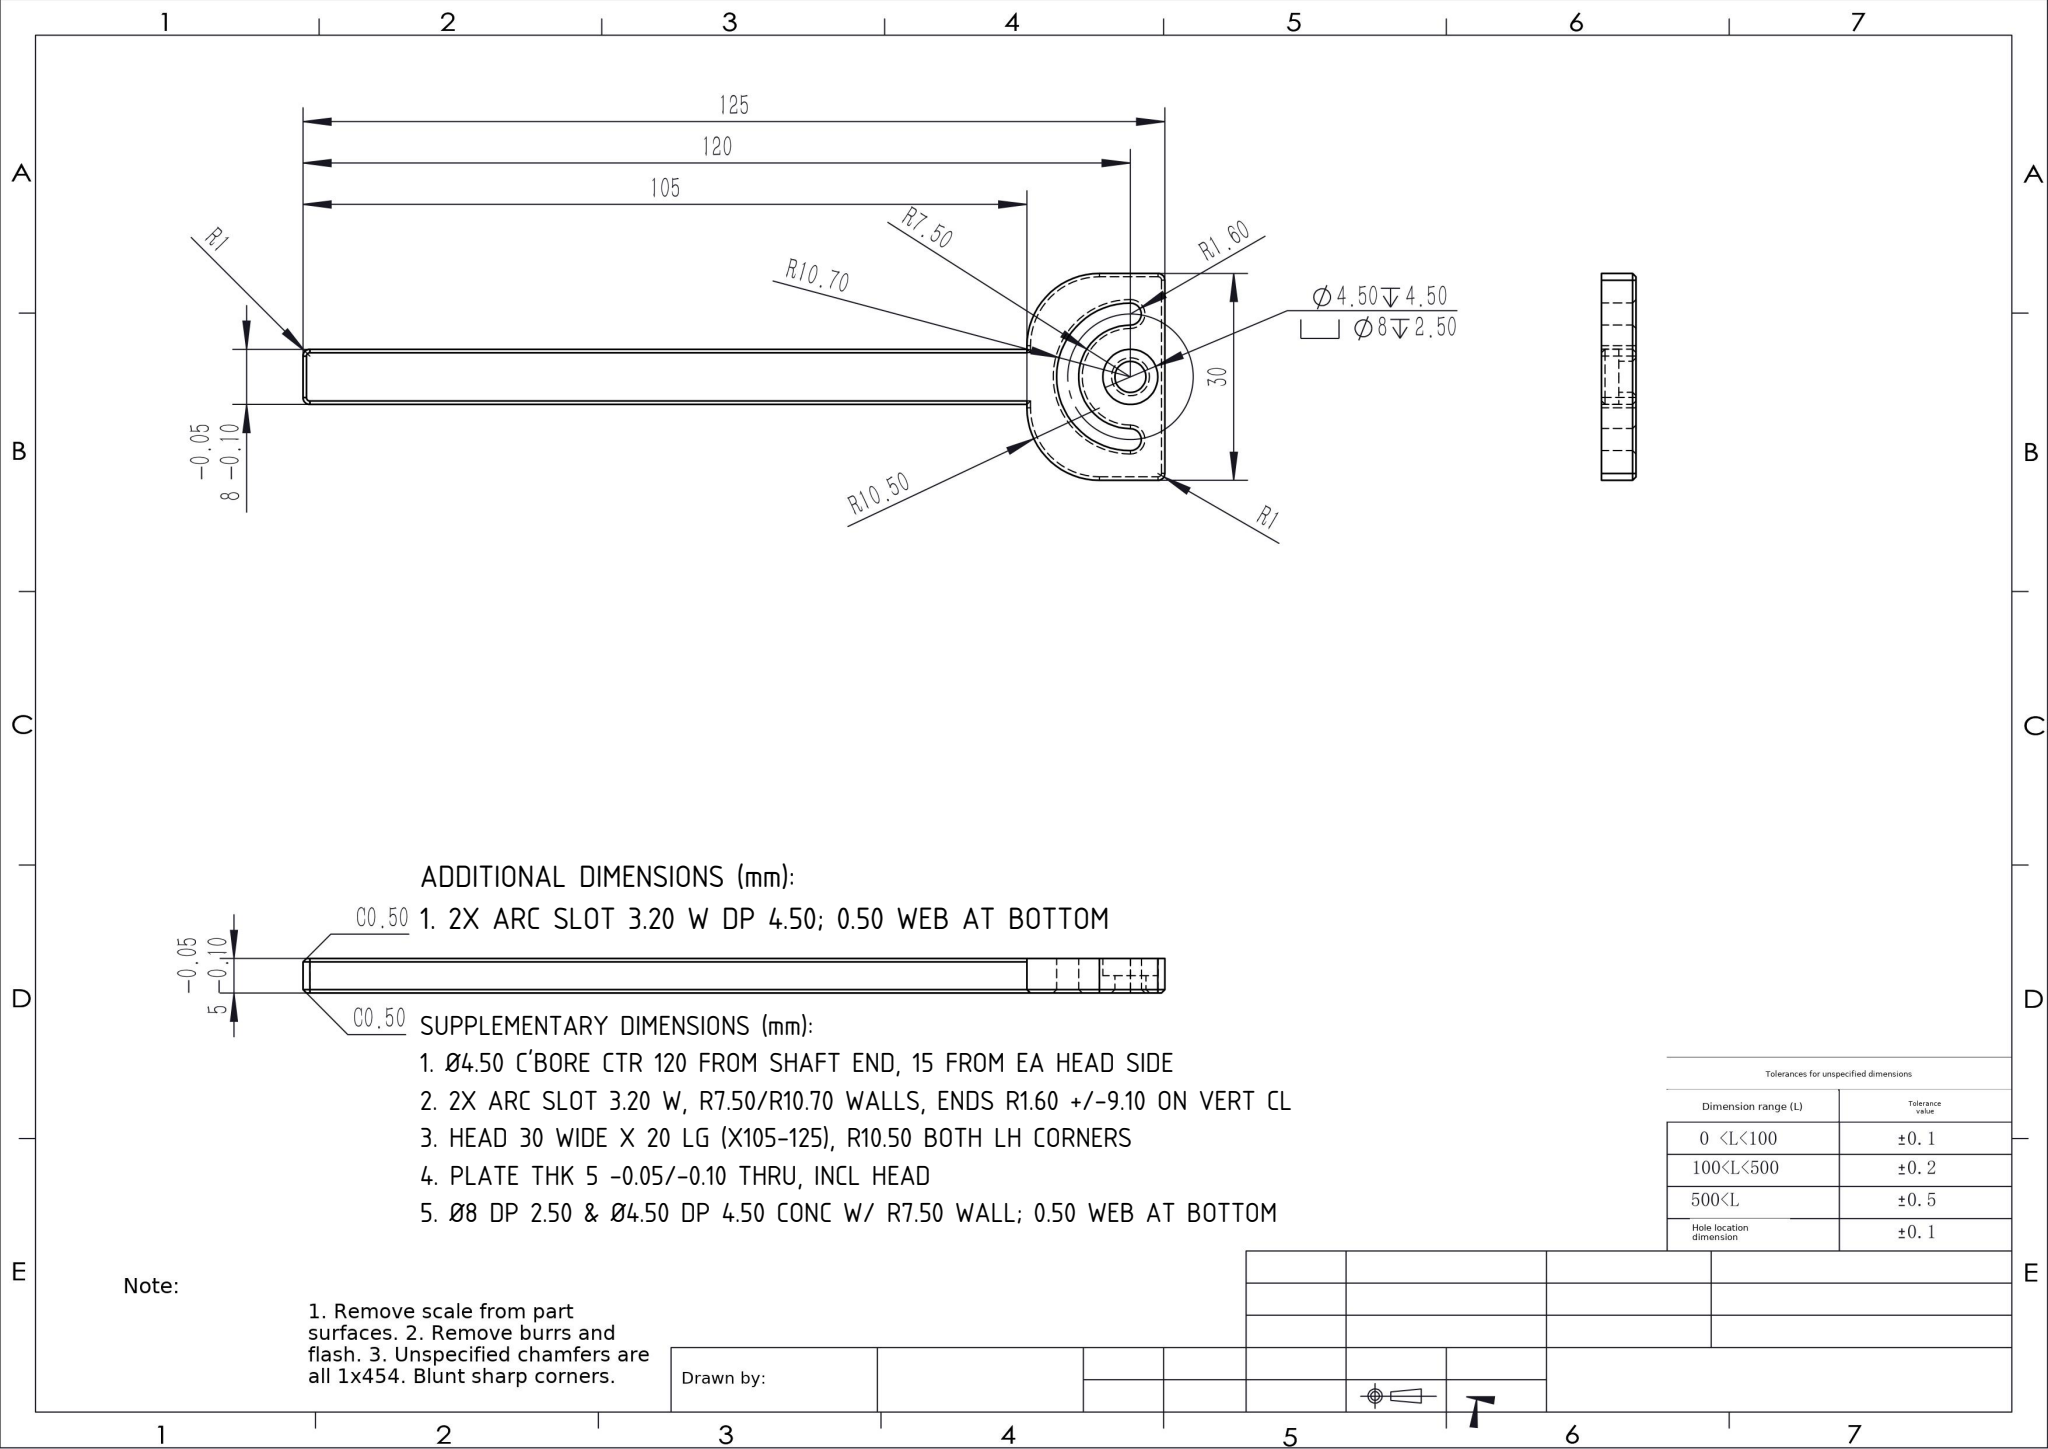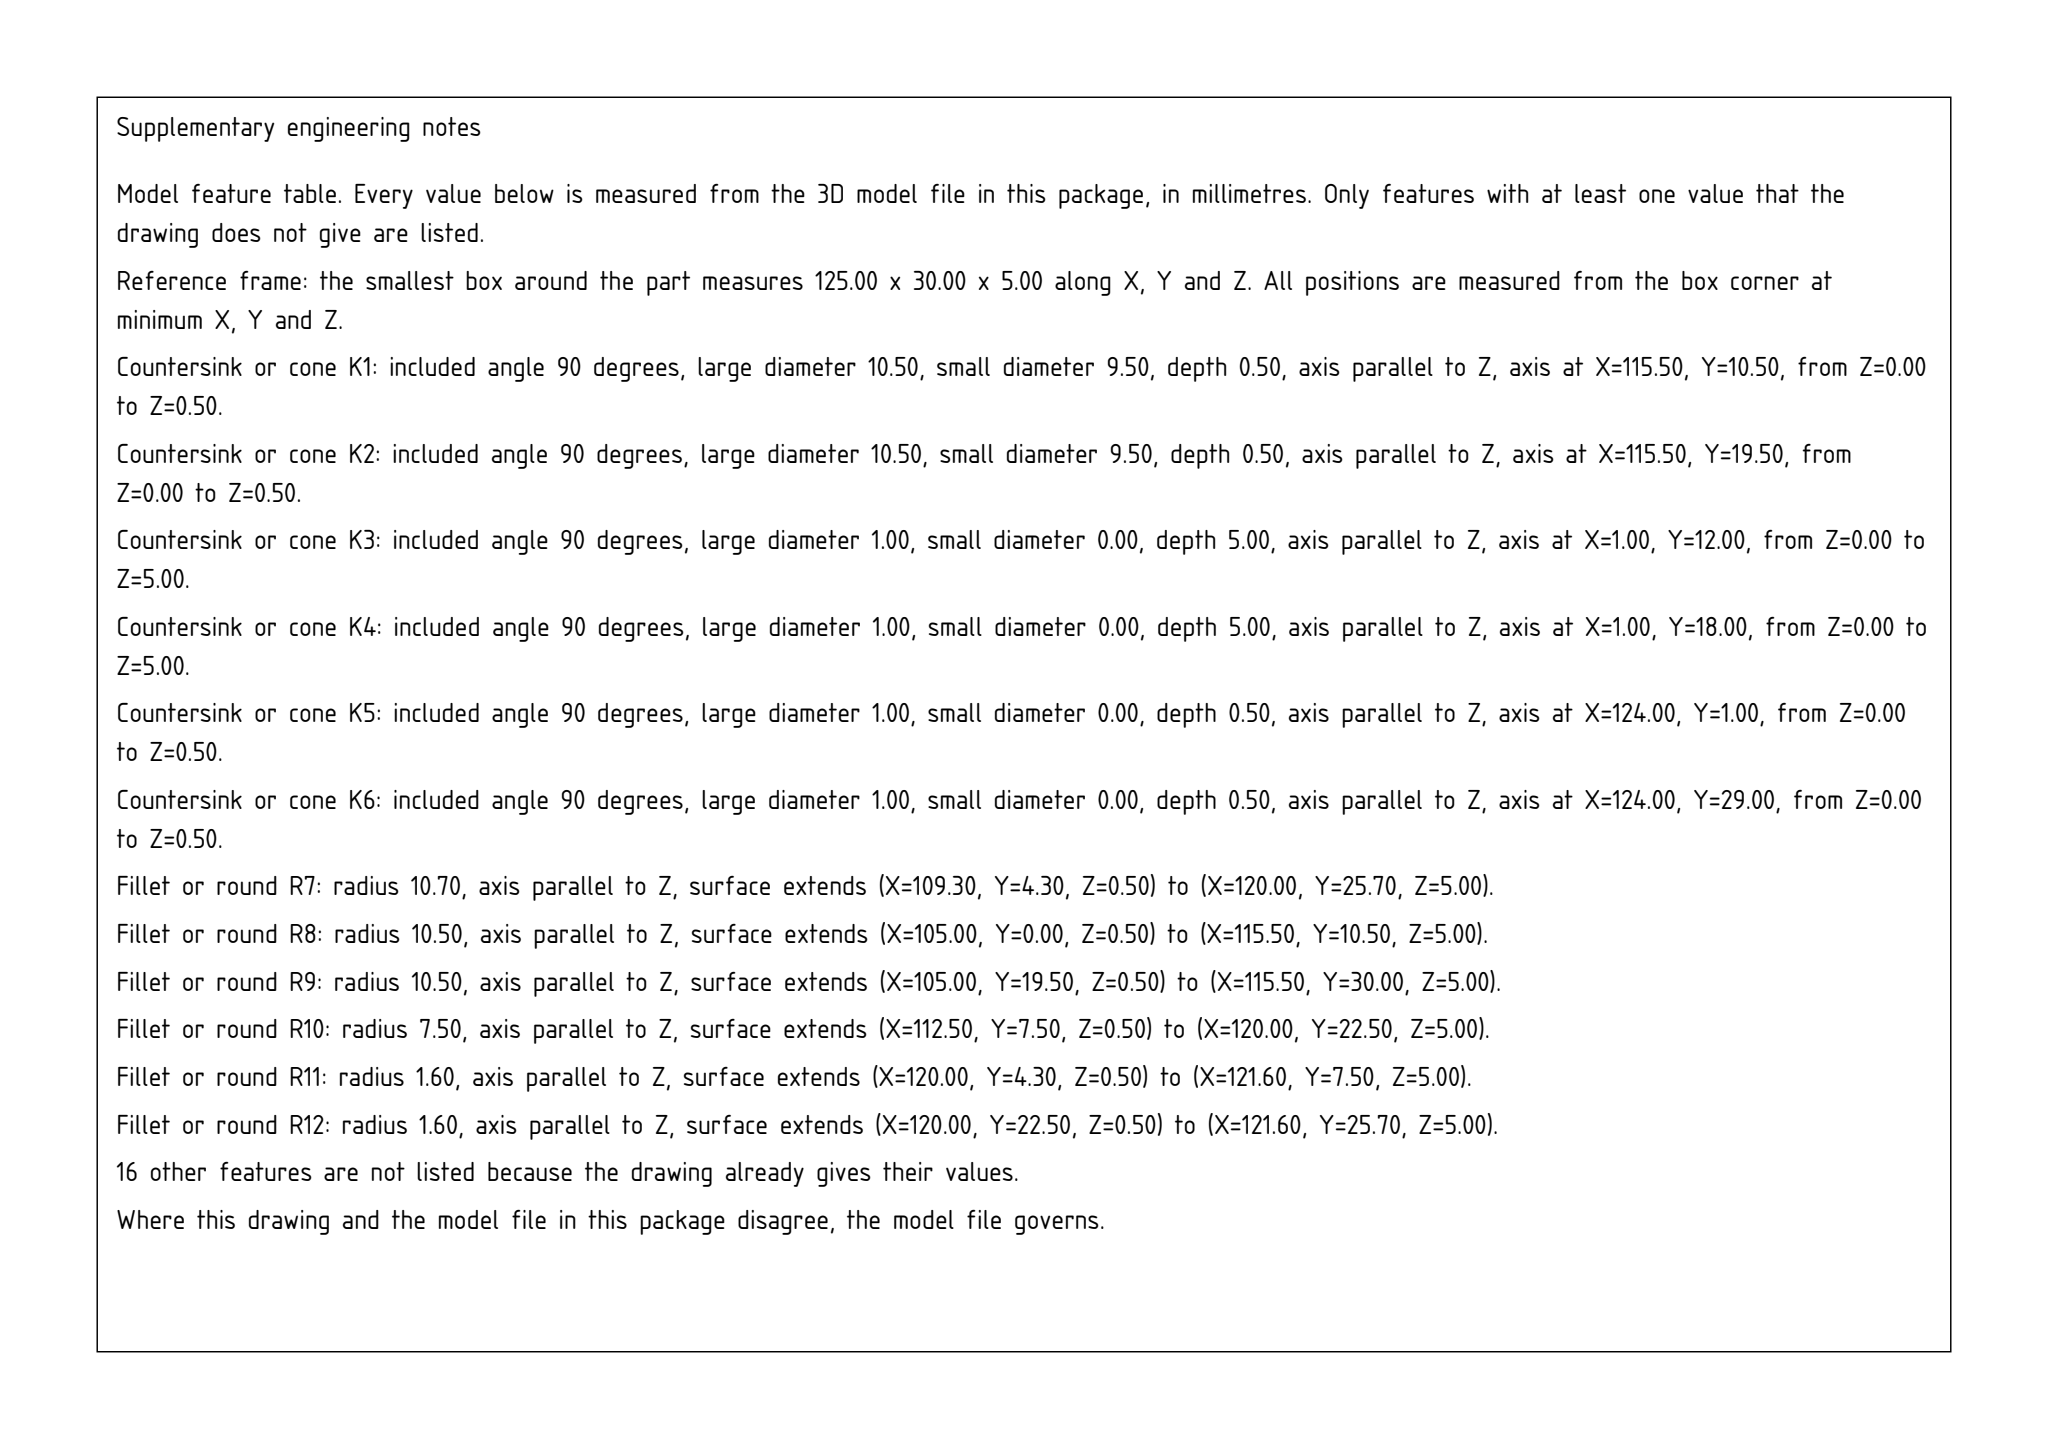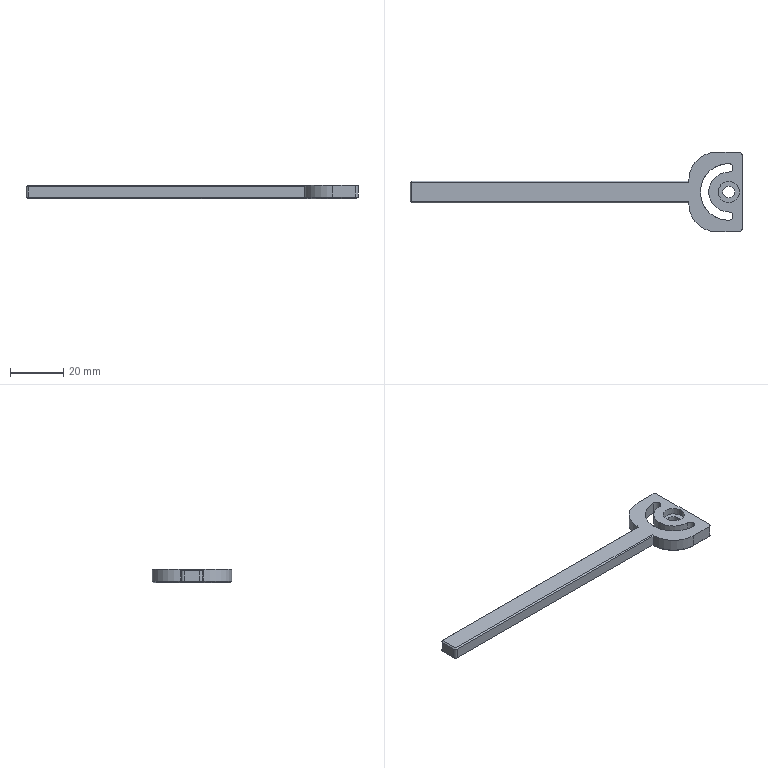Part | SolidWorks | mm | 1 solid | 53 faces | box 125 x 30 x 5 mm | volume 6221 mm3 | plane 22 | cylinder 16 | cone 15 | commonest cylinder face diameters 3.2 x4 2 x4 8 x2 4.5 x2 21 x2 15 x1 21.4 x1
build123d program:
from build123d import *

# Parameters (mm, degrees)
SKETCH2_W           = 105
SKETCH2_H           = 8
BOSS_EXTRUDE1_DEPTH = 5
SKETCH3_R           = 2.25
BOSS_EXTRUDE2_DEPTH = 5
FILLET1_R           = 1
FILLET2_R           = 1
CHAMFER1_SIZE       = 0.5
SKETCH4_R           = 4
CUT_EXTRUDE1_DEPTH  = 2.5


with BuildPart() as part:
    # Sketch2 → Boss-Extrude1 (new body)
    with BuildSketch(Plane.XY):
        Rectangle(SKETCH2_W, SKETCH2_H)
    extrude(amount=BOSS_EXTRUDE1_DEPTH)

    # Sketch3 → Boss-Extrude2 (add)
    with BuildSketch(Plane.XY.offset(5)):
        with BuildLine():
            Line((63, -15), (72.5, -15))
            Line((72.5, -15), (72.5, 15))
            Line((72.5, 15), (63, 15))
            ThreePointArc((63, 15), (55.575, 11.925), (52.5, 4.5))
            Line((52.5, 4.5), (52.5, -4.5))
            ThreePointArc((52.5, -4.5), (55.575, -11.925), (63, -15))
        make_face()
        with Locations((67.5, 0)):
            Circle(SKETCH3_R, mode=Mode.SUBTRACT)
        with BuildLine():
            ThreePointArc((67.5, 7.5), (60, 0), (67.5, -7.5))
            ThreePointArc((67.5, -7.5), (69.1, -9.1), (67.5, -10.7))
            ThreePointArc((67.5, -10.7), (56.8, 0), (67.5, 10.7))
            ThreePointArc((67.5, 10.7), (69.1, 9.1), (67.5, 7.5))
        make_face(mode=Mode.SUBTRACT)
    extrude(amount=-BOSS_EXTRUDE2_DEPTH)

    # Fillet1
    fillet1_edges = [part.edges().sort_by_distance(p)[0] for p in [
        (72.5, 15, 2.5),
        (72.5, -15, 2.5),
    ]]
    fillet(fillet1_edges, radius=FILLET1_R)

    # Fillet2
    fillet2_edges = [part.edges().sort_by_distance(p)[0] for p in [
        (-52.5, -4, 2.5),
        (-52.5, 4, 2.5),
    ]]
    fillet(fillet2_edges, radius=FILLET2_R)

    # Chamfer1
    chamfer1_edges = [part.edges().sort_by_distance(p)[0] for p in [
        (52.5, 4.25, 0),
        (52.5, -4.25, 0),
        (67.25, -15, 0),
        (55.575, -11.925, 0),
        (55.575, 11.925, 0),
        (69.1, 9.1, 0),
        (56.8, 0, 0),
        (69.1, -9.1, 0),
        (60, 0, 0),
        (65.25, 0, 0),
        (72.5, 0, 0),
        (67.25, 15, 0),
        (72.207, 14.707, 0),
        (72.207, -14.707, 0),
        (0.5, 4, 0),
        (-52.5, 0, 0),
        (-52.5, 0, 5),
        (0.5, -4, 0),
        (-52.207, -3.707, 0),
        (-52.207, 3.707, 0),
        (0.5, -4, 5),
        (-52.207, -3.707, 5),
        (-52.207, 3.707, 5),
        (0.5, 4, 5),
    ]]
    chamfer(chamfer1_edges, length=CHAMFER1_SIZE)

    # Sketch4 → Cut-Extrude1 (cut)
    with BuildSketch(Plane.XY.offset(5)):
        with Locations((67.5, 0)):
            Circle(SKETCH4_R)
    extrude(amount=-CUT_EXTRUDE1_DEPTH, mode=Mode.SUBTRACT)


solid = part.part